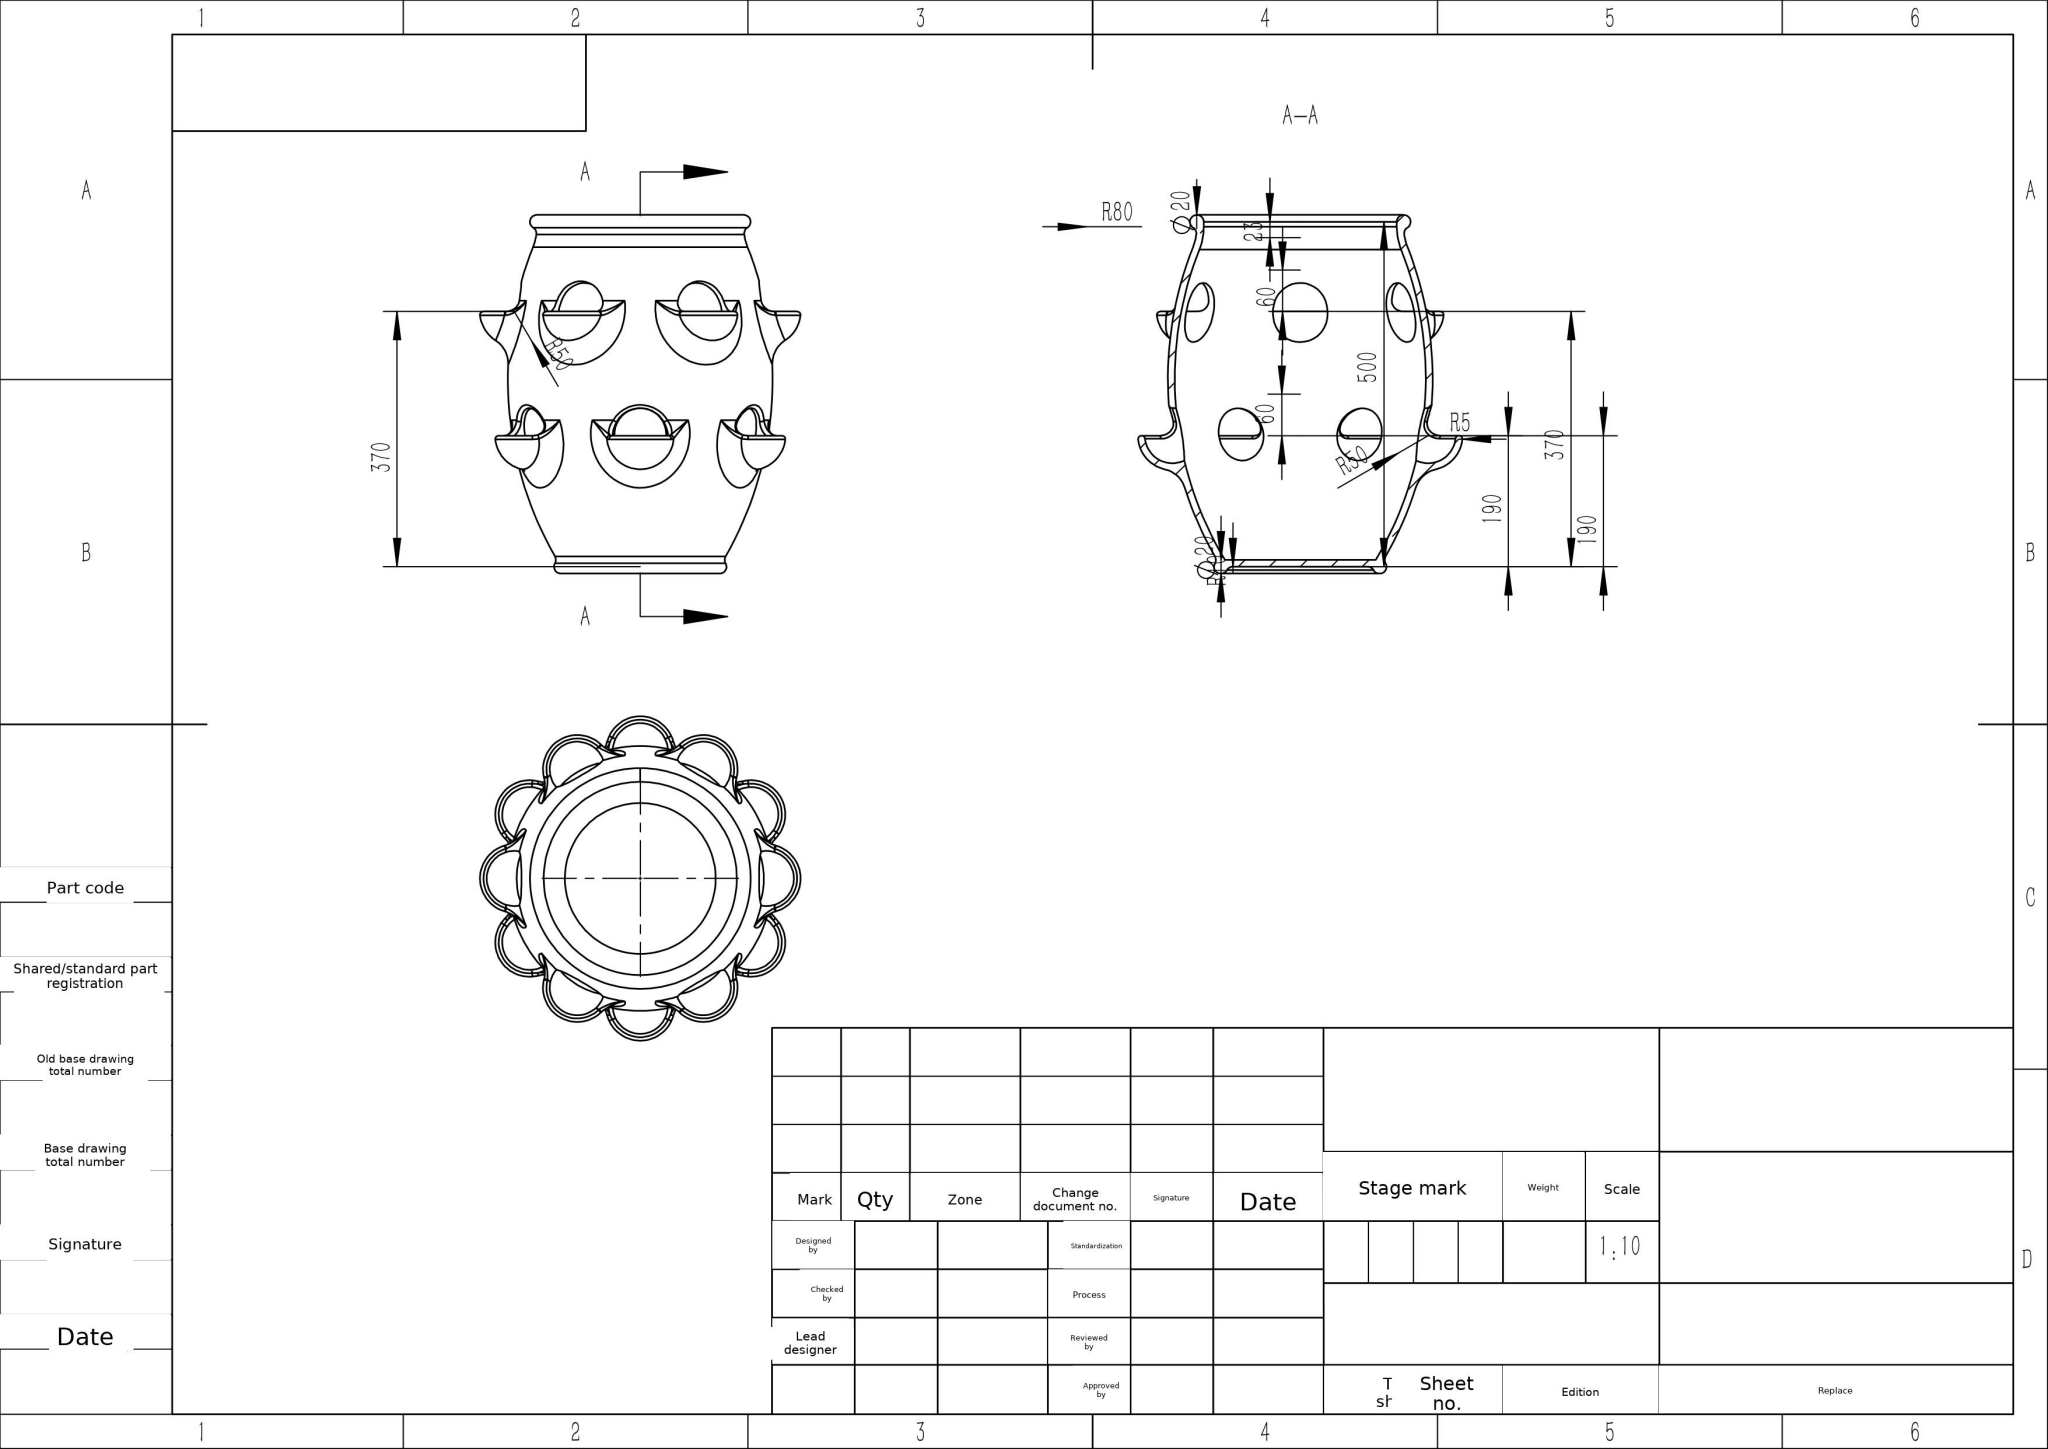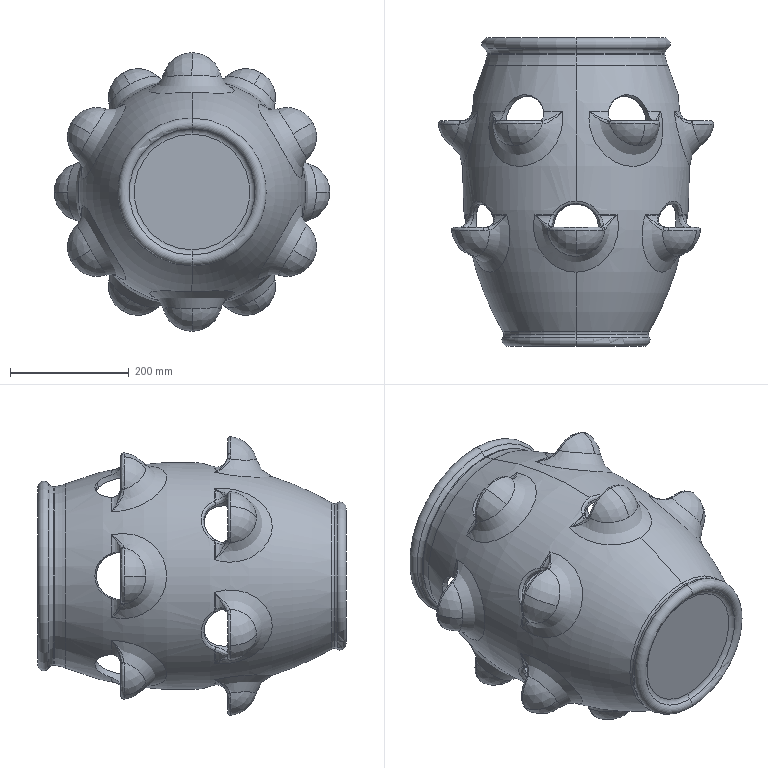Part | SolidWorks | mm | 1 solid | 224 faces | box 464.9 x 520 x 470.32 mm | volume 6550127 mm3 | torus 88 | spline 78 | sphere 48 | plane 8 | cylinder 2 | commonest cylinder face diameters 280 x2